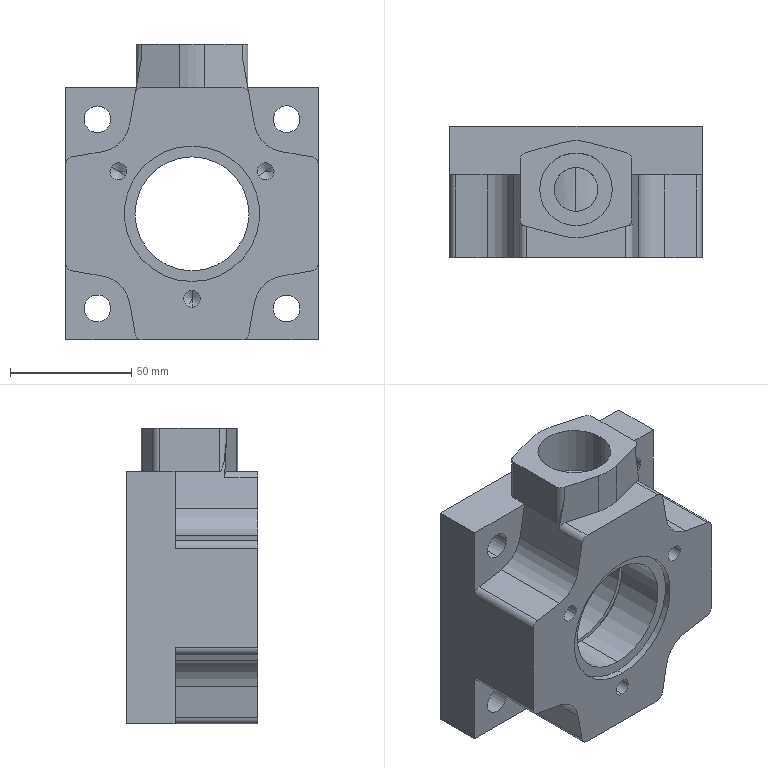Component | SolidWorks | 7-1 | 1 solid | 98 faces | box 104 x 54 x 122 mm | volume 320955 mm3 | cylinder 56 | plane 36 | cone 6 | commonest cylinder face diameters 6 x12 11 x8 7 x6 47 x4 18 x4 27 x4 30 x2 72 x2
build123d program:
from build123d import *

# Parameters (mm, degrees)
SKETCH1_W                = 104
SKETCH1_H                = 104
BOSS_EXTRUDE1_DEPTH      = 20
BOSS_EXTRUDE2_DEPTH      = 34
BOSS_EXTRUDE3_DEPTH      = 18
FILLET1_R                = 3
SKETCH7_R                = 27.9
CUT_EXTRUDE1_DEPTH       = 2.75
CIRPATTERN1_COUNT        = 3
SKETCH8_R                = 23.5
CUT_EXTRUDE2_DEPTH       = 21.05
SKETCH9_R                = 25.25
CUT_EXTRUDE3_DEPTH       = 1.5
SKETCH10_R               = 23.5
CUT_EXTRUDE4_DEPTH       = 15
SKETCH12_R               = 44.8
CUT_EXTRUDE5_DEPTH       = 2.75
SKETCH13_R               = 40
CUT_EXTRUDE6_DEPTH       = 9.75
SKETCH14_R               = 36
SKETCH14_R_2             = 27
CUT_EXTRUDE7_DEPTH       = 15
SKETCH15_R               = 27
CUT_EXTRUDE8_DEPTH       = 1
CUT_EXTRUDE9_START       = -72
SKETCH16_R               = 23.5
CUT_EXTRUDE9_DEPTH       = 72
SKETCH17_R               = 15
CUT_EXTRUDE10_DEPTH      = 20
CUT_EXTRUDE11_REACH      = 128.586
CUT_EXTRUDE11_END_RADIUS = 27
SKETCH18_R               = 9
CUT_EXTRUDE14_DEPTH      = 22
SKETCH20_R               = 5.5
CUT_EXTRUDE15_DEPTH      = 20
CIRPATTERN2_COUNT        = 4
FILLET3_R                = 3


with BuildPart() as part:
    # Sketch1 → Boss-Extrude1 (new body)
    with BuildSketch(Plane(origin=(0, 0, 0), x_dir=(1, 0, 0), z_dir=(0, 1, 0))):
        Rectangle(SKETCH1_W, SKETCH1_H)
    extrude(amount=BOSS_EXTRUDE1_DEPTH)

    # Sketch2 → Boss-Extrude2 (add)
    with BuildSketch(Plane(origin=(0, 20, 0), x_dir=(1, 0, 0), z_dir=(0, 1, 0))):
        with BuildLine():
            Line((23, 52), (-23, 52))
            Line((-23, 52), (-25.705, 36.656))
            ThreePointArc((-25.705, 36.656), (-29.454, 29.454), (-36.656, 25.705))
            Line((-36.656, 25.705), (-52, 23))
            Line((-52, 23), (-52, -23))
            Line((-52, -23), (-36.656, -25.705))
            ThreePointArc((-36.656, -25.705), (-29.454, -29.454), (-25.705, -36.656))
            Line((-25.705, -36.656), (-23, -52))
            Line((-23, -52), (23, -52))
            Line((23, -52), (25.705, -36.656))
            ThreePointArc((25.705, -36.656), (29.454, -29.454), (36.656, -25.705))
            Line((36.656, -25.705), (52, -23))
            Line((52, -23), (52, 23))
            Line((52, 23), (36.656, 25.705))
            ThreePointArc((36.656, 25.705), (29.454, 29.454), (25.705, 36.656))
            Line((25.705, 36.656), (23, 52))
        make_face()
    extrude(amount=BOSS_EXTRUDE2_DEPTH)

    # Sketch3 → Boss-Extrude3 (add)
    with BuildSketch(Plane(origin=(0, 0, -52), x_dir=(-1, 0, 0), z_dir=(0, 0, -1))):
        with BuildLine():
            Line((5.176, 6.681), (23, 11.457))
            Line((23, 11.457), (23, 40.543))
            Line((23, 40.543), (5.176, 45.319))
            ThreePointArc((5.176, 45.319), (0, 46), (-5.176, 45.319))
            Line((-5.176, 45.319), (-23, 40.543))
            Line((-23, 40.543), (-23, 11.457))
            Line((-23, 11.457), (-5.176, 6.681))
            ThreePointArc((-5.176, 6.681), (0, 6), (5.176, 6.681))
        make_face()
    extrude(amount=BOSS_EXTRUDE3_DEPTH)

    # Fillet1
    fillet1_edges = [part.edges().sort_by_distance(p)[0] for p in [
        (-52, 37, 23),
        (-23, 37, 52),
        (23, 37, 52),
        (52, 37, 23),
        (52, 37, -23),
        (23, 47.271, -52),
        (-23, 47.271, -52),
        (-52, 37, -23),
    ]]
    fillet(fillet1_edges, radius=FILLET1_R)

    # Sketch7 → Cut-Extrude1 (cut)
    with BuildSketch(Plane(origin=(0, 54, 0), x_dir=(1, 0, 0), z_dir=(0, 1, 0))):
        with Locations(Location((0, 0, 0), (0, 0, 270))):
            Circle(SKETCH7_R)
    extrude(amount=-CUT_EXTRUDE1_DEPTH, mode=Mode.SUBTRACT)

    # Sketch6 → Size mm Dowel Pin Hole1 (revolve, cut)
    with BuildSketch(Plane(origin=(0, 54, 35), x_dir=(0, 0, 1), z_dir=(1, 0, 0))):
        Polygon((0, 0), (0, 18.021), (3.5, 16), (3.5, 0), align=None)
    size_mm_dowel_pin_hole1 = revolve(axis=Axis((0, 60.35, 35), (0, -1, 0)), mode=Mode.SUBTRACT)

    # CirPattern1: Size mm Dowel Pin Hole1 ×3 about axis
    cirpattern1_axis = Axis((0, 0, 0), (0, 1, 0))
    for i in range(1, CIRPATTERN1_COUNT):
        add(size_mm_dowel_pin_hole1.rotate(cirpattern1_axis, i * 360 / CIRPATTERN1_COUNT), mode=Mode.SUBTRACT)

    # Sketch8 → Cut-Extrude2 (cut)
    with BuildSketch(Plane(origin=(0, 51.25, 0), x_dir=(1, 0, 0), z_dir=(0, 1, 0))):
        with Locations(Location((0, 0, 0), (0, 0, 270))):
            Circle(SKETCH8_R)
    extrude(amount=-CUT_EXTRUDE2_DEPTH, mode=Mode.SUBTRACT)

    # Sketch9 → Cut-Extrude3 (cut)
    with BuildSketch(Plane(origin=(0, 30.2, 0), x_dir=(1, 0, 0), z_dir=(0, 1, 0))):
        with Locations(Location((0, 0, 0), (0, 0, 270))):
            Circle(SKETCH9_R)
    extrude(amount=-CUT_EXTRUDE3_DEPTH, mode=Mode.SUBTRACT)

    # Sketch10 → Cut-Extrude4 (cut)
    with BuildSketch(Plane(origin=(0, 28.7, 0), x_dir=(1, 0, 0), z_dir=(0, 1, 0))):
        with Locations(Location((0, 0, 0), (0, 0, 270))):
            Circle(SKETCH10_R)
    extrude(amount=-CUT_EXTRUDE4_DEPTH, mode=Mode.SUBTRACT)

    # Sketch12 → Cut-Extrude5 (cut)
    with BuildSketch(Plane.XZ):
        with Locations(Location((0, 0, 0), (0, 0, 270))):
            Circle(SKETCH12_R)
    extrude(amount=-CUT_EXTRUDE5_DEPTH, mode=Mode.SUBTRACT)

    # Sketch13 → Cut-Extrude6 (cut)
    with BuildSketch(Plane.XZ.offset(-2.75)):
        with Locations(Location((0, 0, 0), (0, 0, 270))):
            Circle(SKETCH13_R)
    extrude(amount=-CUT_EXTRUDE6_DEPTH, mode=Mode.SUBTRACT)

    # Sketch14 → Cut-Extrude7 (cut)
    with BuildSketch(Plane.XZ.offset(-12.5)):
        with Locations(Location((0, 0, 0), (0, 0, 270))):
            Circle(SKETCH14_R)
        with Locations(Location((0, 0, 0), (0, 0, 270))):
            Circle(SKETCH14_R_2, mode=Mode.SUBTRACT)
    extrude(amount=-CUT_EXTRUDE7_DEPTH, mode=Mode.SUBTRACT)

    # Sketch15 → Cut-Extrude8 (cut)
    with BuildSketch(Plane.XZ.offset(-12.5)):
        with Locations(Location((0, 0, 0), (0, 0, 270))):
            Circle(SKETCH15_R)
    extrude(amount=-CUT_EXTRUDE8_DEPTH, mode=Mode.SUBTRACT)

    # Sketch16 → Cut-Extrude9 (cut)
    with BuildSketch(Plane.XZ.offset(-13.5).offset(CUT_EXTRUDE9_START)):
        with Locations(Location((0, 0, 0), (0, 0, 90))):
            Circle(SKETCH16_R)
    extrude(amount=CUT_EXTRUDE9_DEPTH, mode=Mode.SUBTRACT)

    # Sketch17 → Cut-Extrude10 (cut)
    with BuildSketch(Plane(origin=(0, 0, -70), x_dir=(-1, 0, 0), z_dir=(0, 0, -1))):
        with Locations((0, 26)):
            Circle(SKETCH17_R)
    extrude(amount=-CUT_EXTRUDE10_DEPTH, mode=Mode.SUBTRACT)

    # Cut-Extrude11: up to this cylinder (the profile starts outside it)
    cut_extrude11_end = Plane(origin=(0, 26, 0), z_dir=(0, -1, 0)) * Cylinder(CUT_EXTRUDE11_END_RADIUS, 312.172, mode=Mode.PRIVATE)
    # Sketch18 → Cut-Extrude11 (cut, up to the surface)
    with BuildSketch(Plane(origin=(0, 0, -50), x_dir=(-1, 0, 0), z_dir=(0, 0, -1)), mode=Mode.PRIVATE) as cut_extrude11_sk1:
        with Locations((0, 26)):
            Circle(SKETCH18_R)
    cut_extrude11_tool1 = extrude(cut_extrude11_sk1.sketch, amount=-CUT_EXTRUDE11_REACH, mode=Mode.PRIVATE) - cut_extrude11_end
    add(cut_extrude11_tool1.solids().sort_by_distance((0, 26, -50))[0], mode=Mode.SUBTRACT)

    # Sketch19 → Cut-Extrude14 (cut)
    with BuildSketch(Plane.XZ.offset(-12.5)):
        with BuildLine():
            ThreePointArc((-9.714, -34.665), (0, -36), (9.714, -34.665))
            ThreePointArc((9.714, -34.665), (12.833, -29.117), (7.286, -25.998))
            ThreePointArc((7.286, -25.998), (0, -27), (-7.286, -25.998))
            ThreePointArc((-7.286, -25.998), (-12.833, -29.117), (-9.714, -34.665))
        make_face()
    extrude(amount=-CUT_EXTRUDE14_DEPTH, mode=Mode.SUBTRACT)

    # Sketch20 → Cut-Extrude15 (cut)
    with BuildSketch(Plane.XZ):
        with Locations(Location((-39, -39, 0), (0, 0, 270))):
            Circle(SKETCH20_R)
    cut_extrude15 = extrude(amount=-CUT_EXTRUDE15_DEPTH, mode=Mode.SUBTRACT)

    # CirPattern2: Cut-Extrude15 ×4 about axis
    cirpattern2_axis = Axis((0, 0, 0), (0, 1, 0))
    for i in range(1, CIRPATTERN2_COUNT):
        add(cut_extrude15.rotate(cirpattern2_axis, i * 360 / CIRPATTERN2_COUNT), mode=Mode.SUBTRACT)

    # Fillet3
    fillet3_edges = [part.edges().sort_by_distance(p)[0] for p in [
        (-23, 11.457, -61),
        (-23, 40.543, -61),
        (23, 40.543, -61),
        (23, 11.457, -61),
    ]]
    fillet(fillet3_edges, radius=FILLET3_R)


solid = part.part

# Placed as in the assembly
solid = solid.moved(Location((0, -20.881, 0), (180, 0, 0)))